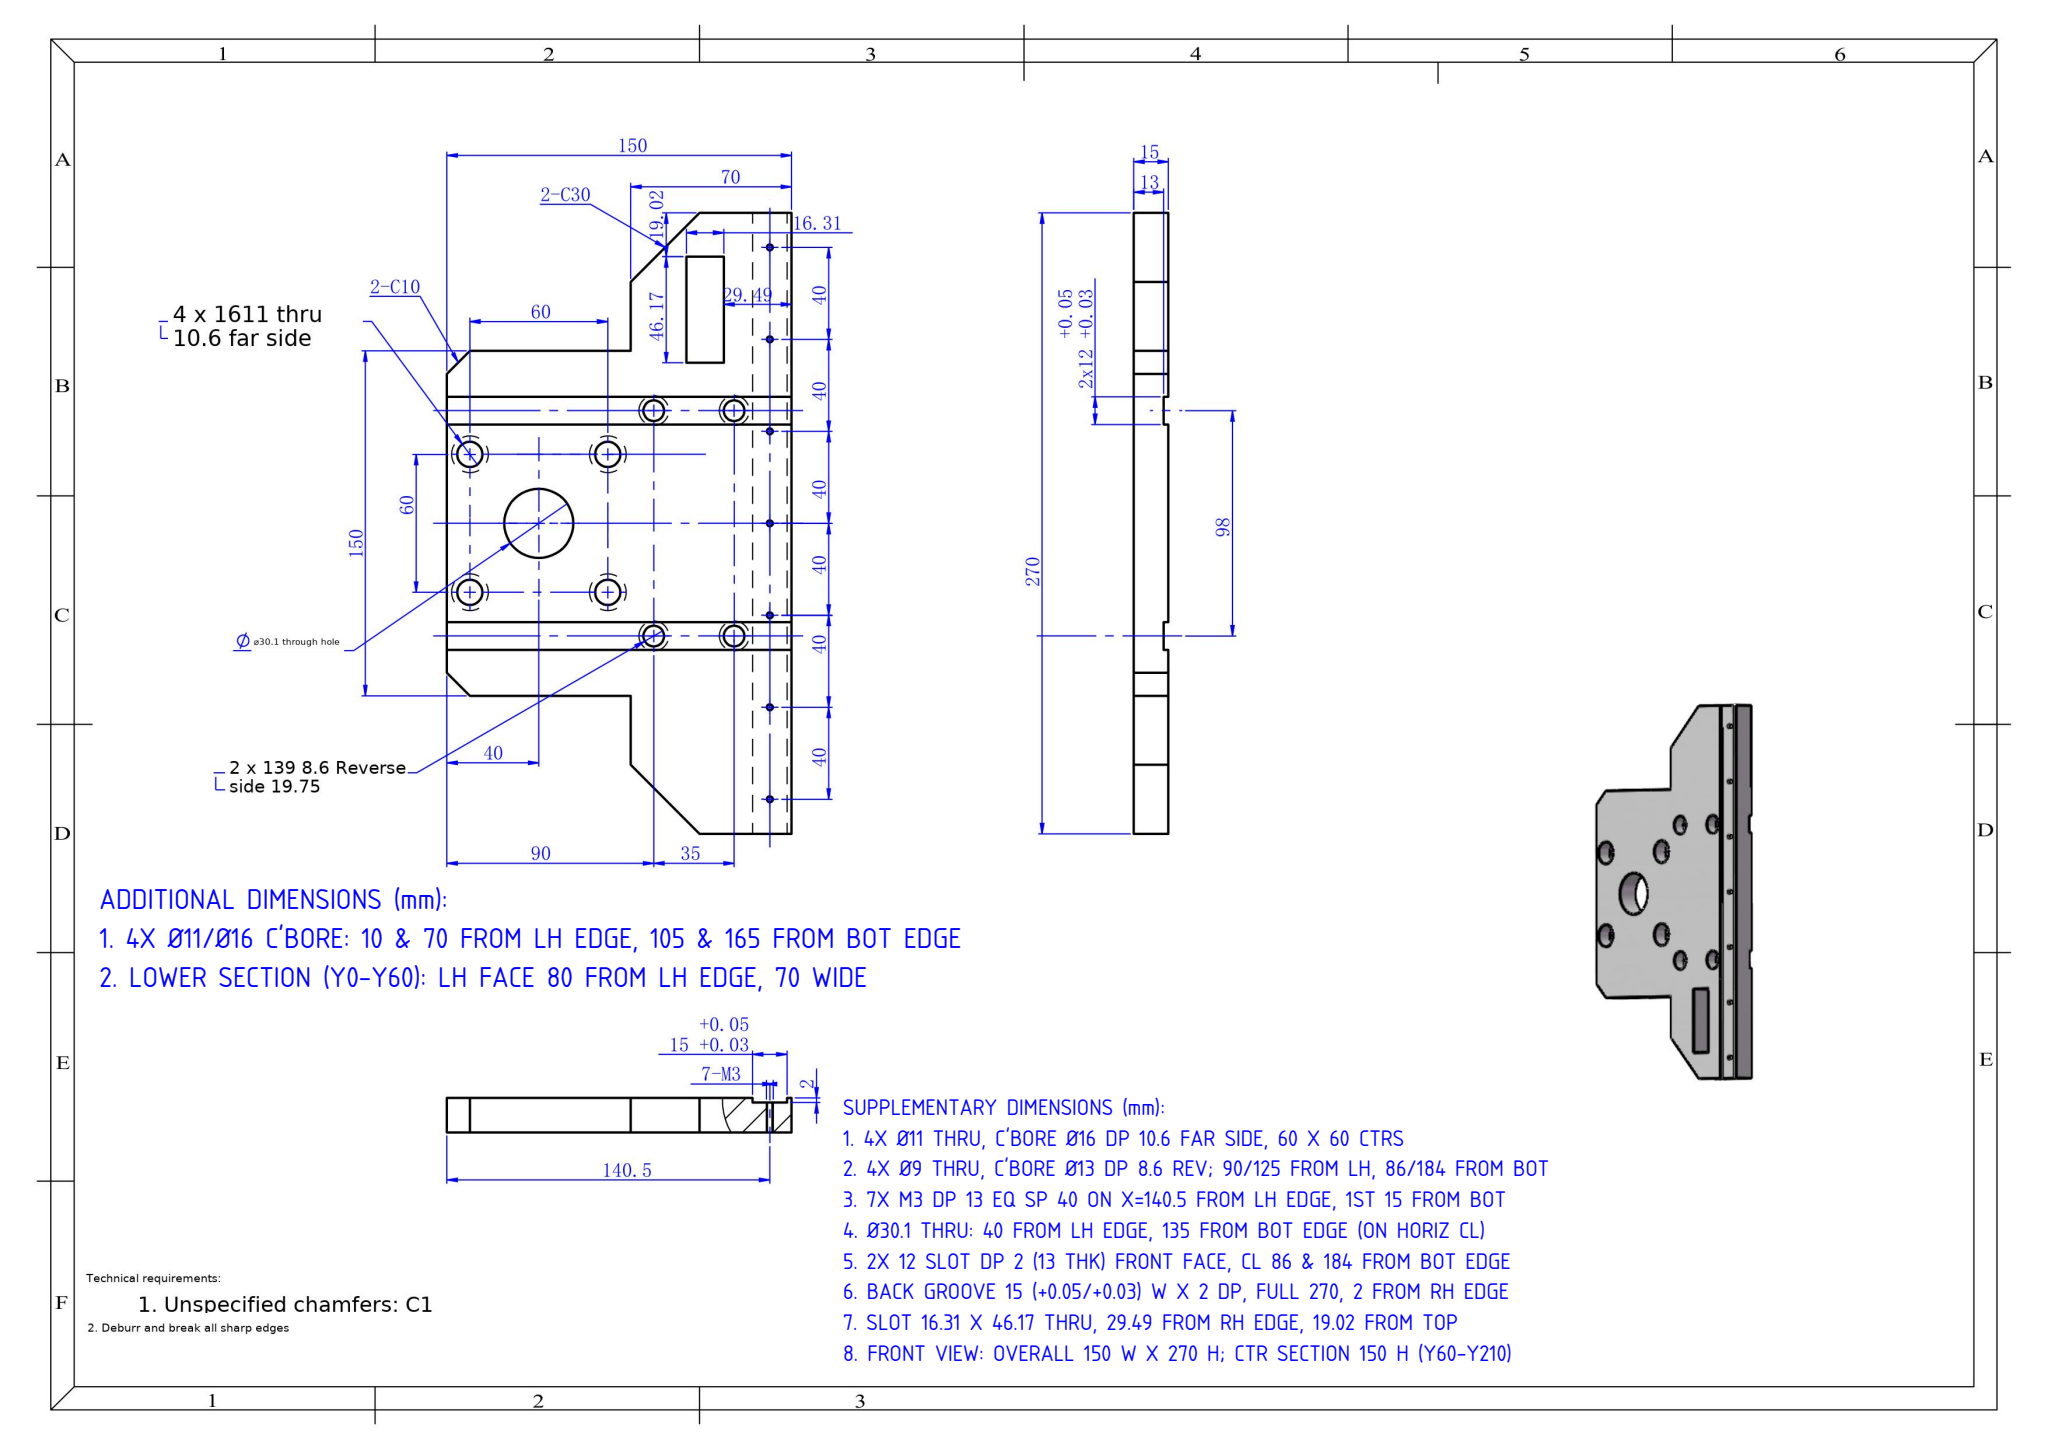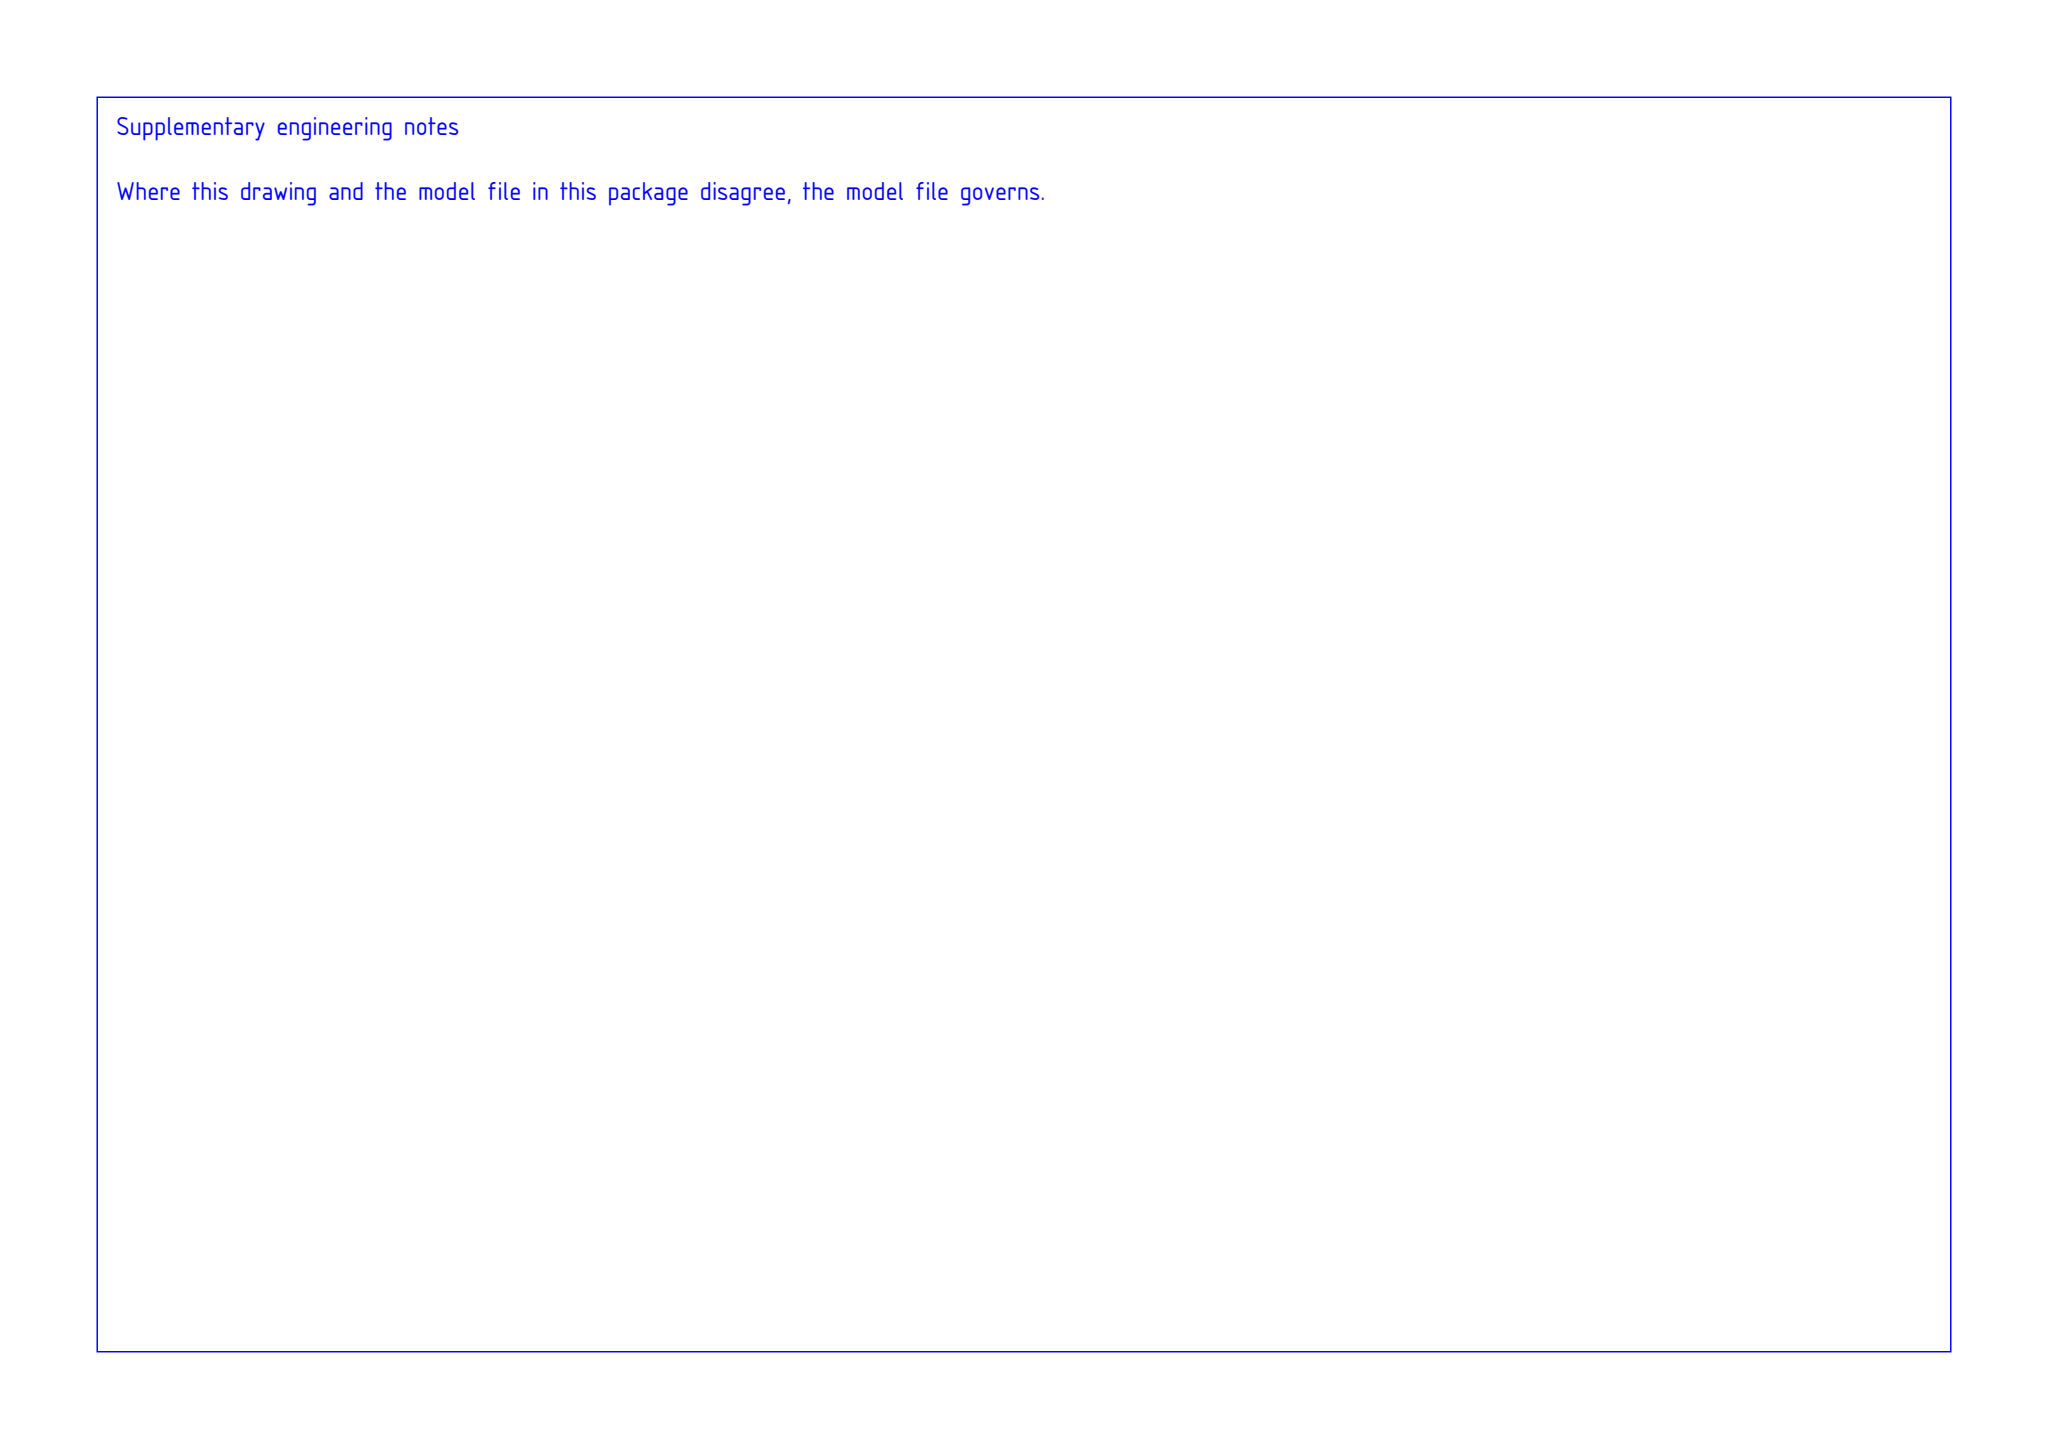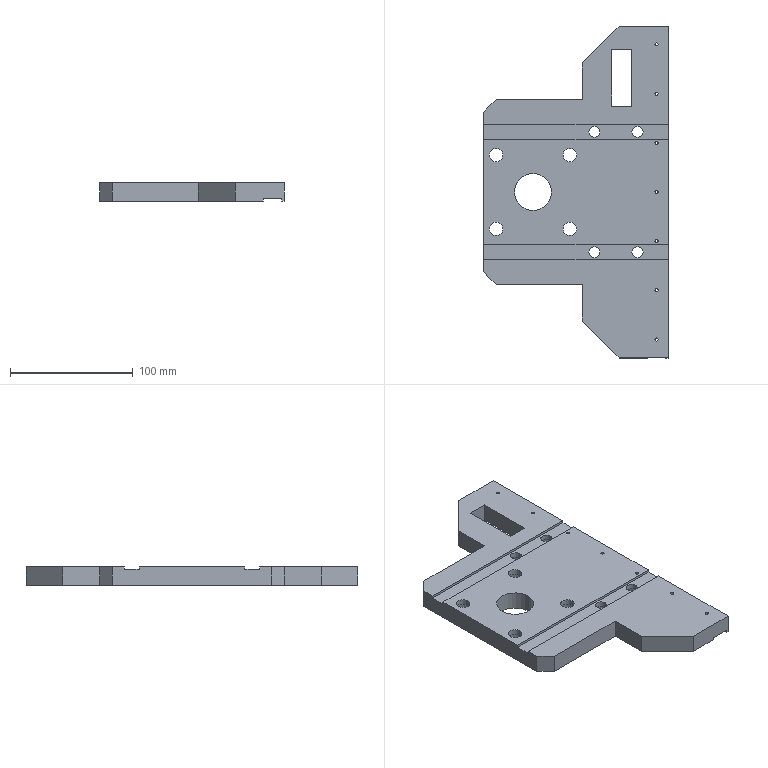Part | SolidWorks | mm | 1 solid | 86 faces | box 150 x 270 x 15 mm | volume 394899 mm3 | cylinder 48 | plane 38 | commonest cylinder face diameters 2.5 x14 13 x8 9 x8 16 x8 11 x8 30.1 x2
build123d program:
from build123d import *

# Parameters (mm, degrees)
SKETCH1_W                                        = 150
SKETCH1_H                                        = 270
BOSS_EXTRUDE1_DEPTH                              = 15
SKETCH2_W                                        = 15
SKETCH2_H                                        = 2
CUT_EXTRUDE1_DEPTH                               = 281.958
SKETCH3_R                                        = 15.05
CUT_EXTRUDE2_DEPTH                               = 204.545
M3_TAPPED_HOLE1_D                                = 2.5
M10_HEX_SOCKET_HEAD_CAP_SCREW_CBORE1_D           = 11
M10_HEX_SOCKET_HEAD_CAP_SCREW_CBORE1_CBORE_D     = 16
M10_HEX_SOCKET_HEAD_CAP_SCREW_CBORE1_CBORE_DEPTH = 10.6
SKETCH8_W                                        = 2
SKETCH8_H                                        = 12
CUT_EXTRUDE3_DEPTH                               = 242.077
M8_HEX_SOCKET_HEAD_CAP_SCREW_CBORE1_AT_2_COUNT   = 2
M8_HEX_SOCKET_HEAD_CAP_SCREW_CBORE1_AT_2_PITCH   = 35
SKETCH11_W                                       = 80
SKETCH11_H                                       = 60
CUT_EXTRUDE4_DEPTH                               = 204.545
CHAMFER1_SIZE                                    = 30
CHAMFER2_SIZE                                    = 10
SKETCH12_W                                       = 16.312
SKETCH12_H                                       = 46.172
CUT_EXTRUDE5_DEPTH                               = 136


with BuildPart() as part:
    # Sketch1 → Boss-Extrude1 (new body)
    with BuildSketch(Plane.XY):
        with Locations((-1.239, -53.13)):
            Rectangle(SKETCH1_W, SKETCH1_H)
    extrude(amount=BOSS_EXTRUDE1_DEPTH)

    # Sketch2 → Cut-Extrude1 (cut, through all)
    with BuildSketch(Plane(origin=(0, 81.87, 0), x_dir=(1, 0, 0), z_dir=(0, 1, 0))):
        with Locations((64.261, -1)):
            Rectangle(SKETCH2_W, SKETCH2_H)
    extrude(amount=-CUT_EXTRUDE1_DEPTH, mode=Mode.SUBTRACT)

    # Sketch3 → Cut-Extrude2 (cut, through all)
    with BuildSketch(Plane(origin=(0, 0, 0), x_dir=(-1, 0, 0), z_dir=(0, 0, -1))):
        with Locations((36.239, -53.13)):
            Circle(SKETCH3_R)
    extrude(amount=-CUT_EXTRUDE2_DEPTH, mode=Mode.SUBTRACT)

    # M3 Tapped Hole1 (through all)
    with Locations(Plane(origin=(0, 0, 2), x_dir=(-1, 0, 0), z_dir=(0, 0, -1))):
        with Locations((-64.261, -173.13), (-64.261, -133.13), (-64.261, -93.13), (-64.261, -53.13), (-64.261, -13.13), (-64.261, 26.87), (-64.261, 66.87)):
            Hole(M3_TAPPED_HOLE1_D / 2)

    # M10 Hex Socket Head Cap Screw CBORE1 (through all)
    with Locations(Plane(origin=(0, 0, 0), x_dir=(-1, 0, 0), z_dir=(0, 0, -1))):
        with Locations((66.239, -23.13), (66.239, -83.13), (6.239, -83.13), (6.239, -23.13)):
            CounterBoreHole(M10_HEX_SOCKET_HEAD_CAP_SCREW_CBORE1_D / 2, M10_HEX_SOCKET_HEAD_CAP_SCREW_CBORE1_CBORE_D / 2, M10_HEX_SOCKET_HEAD_CAP_SCREW_CBORE1_CBORE_DEPTH)

    # Sketch8 → Cut-Extrude3 (cut, through all)
    with BuildSketch(Plane(origin=(73.761, 0, 0), x_dir=(0, 0, -1), z_dir=(1, 0, 0))):
        with Locations((-14, -4.13)):
            Rectangle(SKETCH8_W, SKETCH8_H)
    cut_extrude3 = extrude(amount=-CUT_EXTRUDE3_DEPTH, mode=Mode.SUBTRACT)

    # Mirror1: Cut-Extrude3 across plane
    add(cut_extrude3.mirror(Plane.ZX.offset(-53.13)), mode=Mode.SUBTRACT)

    # Sketch10 → M8 Hex Socket Head Cap Screw CBORE1 (revolve, cut)
    with BuildSketch(Plane(origin=(13.761, -4.13, 0), x_dir=(0, 1, 0), z_dir=(1, 0, 0))):
        Polygon((0, 0), (0, 22.454), (4.5, 19.75), (4.5, 8.6), (6.5, 8.6), (6.5, 0), align=None)
    m8_hex_socket_head_cap_screw_cbore1 = revolve(axis=Axis((13.761, -4.13, -6.35), (0, 0, 1)), mode=Mode.SUBTRACT)

    # M8 Hex Socket Head Cap Screw CBORE1 at 2: M8 Hex Socket Head Cap Screw CBORE1 ×2
    with Locations(*[(i * M8_HEX_SOCKET_HEAD_CAP_SCREW_CBORE1_AT_2_PITCH, 0, 0) for i in range(1, M8_HEX_SOCKET_HEAD_CAP_SCREW_CBORE1_AT_2_COUNT)]):
        add(m8_hex_socket_head_cap_screw_cbore1, mode=Mode.SUBTRACT)

    # Mirror2: M8 Hex Socket Head Cap Screw CBORE1 across plane
    add(m8_hex_socket_head_cap_screw_cbore1.mirror(Plane.ZX.offset(-53.13)), mode=Mode.SUBTRACT)

    # Mirror2 copy 1 sketch → Mirror2 copy 1 (revolve, cut)
    with BuildSketch(Plane(origin=(48.761, -102.13, 0), x_dir=(0, -1, 0), z_dir=(1, 0, 0))):
        Polygon((0, 0), (0, -22.454), (4.5, -19.75), (4.5, -8.6), (6.5, -8.6), (6.5, 0), align=None)
    revolve(axis=Axis((48.761, -102.13, -6.35), (0, 0, -1)), mode=Mode.SUBTRACT)

    # Sketch11 → Cut-Extrude4 (cut, through all)
    with BuildSketch(Plane.XY.offset(15)):
        with Locations((-36.239, -158.13)):
            Rectangle(SKETCH11_W, SKETCH11_H)
        with Locations((-36.239, 51.87)):
            Rectangle(SKETCH11_W, SKETCH11_H)
    extrude(amount=-CUT_EXTRUDE4_DEPTH, mode=Mode.SUBTRACT)

    # Chamfer1
    chamfer1_edges = [part.edges().sort_by_distance(p)[0] for p in [
        (3.761, -188.13, 7.5),
        (3.761, 81.87, 7.5),
    ]]
    chamfer(chamfer1_edges, length=CHAMFER1_SIZE)

    # Chamfer2
    chamfer2_edges = [part.edges().sort_by_distance(p)[0] for p in [
        (-76.239, -128.13, 7.5),
        (-76.239, 21.87, 7.5),
    ]]
    chamfer(chamfer2_edges, length=CHAMFER2_SIZE)

    # Sketch12 → Cut-Extrude5 (cut)
    with BuildSketch(Plane(origin=(0, 0, 0), x_dir=(-1, 0, 0), z_dir=(0, 0, -1))):
        with Locations((-36.118, 39.767)):
            Rectangle(SKETCH12_W, SKETCH12_H)
    extrude(amount=-CUT_EXTRUDE5_DEPTH, mode=Mode.SUBTRACT)


solid = part.part